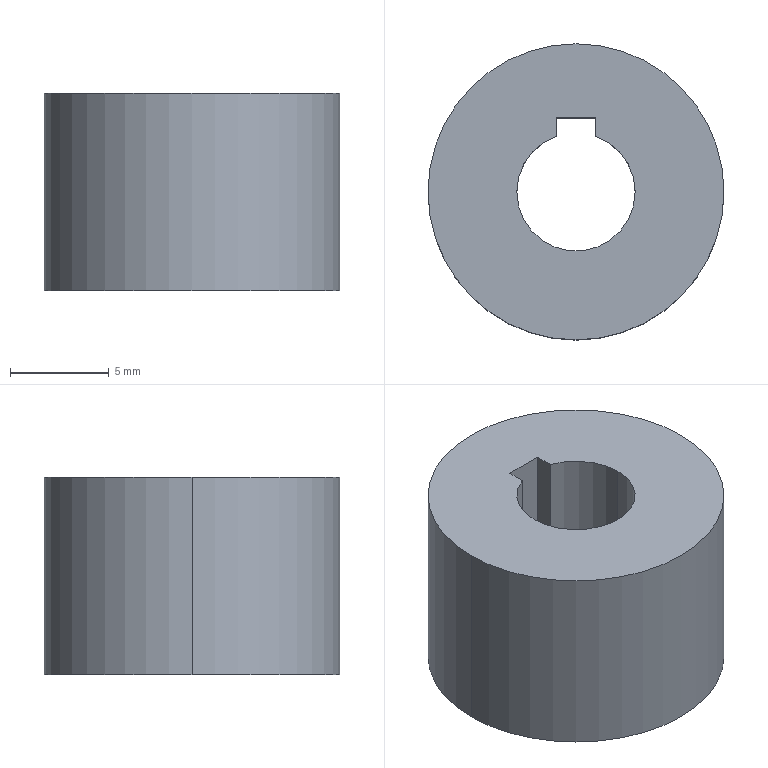Component | SolidWorks | SmallWheel-1 | 1 solid | 10 faces | box 15 x 15 x 10 mm | volume 1468 mm3 | cylinder 5 | plane 5 | commonest cylinder face diameters 6 x3 15 x2
build123d program:
from build123d import *

# Parameters (mm, degrees)
SKETCH1_R           = 7.5
SKETCH1_R_2         = 3
BOSS_EXTRUDE1_DEPTH = 10
SKETCH2_W           = 2
SKETCH2_H           = 1.5
CUT_EXTRUDE1_DEPTH  = 74.46


with BuildPart() as part:
    # Sketch1 → Boss-Extrude1 (new body)
    with BuildSketch(Plane.XY):
        with Locations((59.88, -20)):
            Circle(SKETCH1_R)
        with Locations((59.88, -20)):
            Circle(SKETCH1_R_2, mode=Mode.SUBTRACT)
    extrude(amount=-BOSS_EXTRUDE1_DEPTH)

    # Sketch2 → Cut-Extrude1 (cut, through all)
    with BuildSketch(Plane.XY):
        with Locations((59.88, -17)):
            Rectangle(SKETCH2_W, SKETCH2_H)
    extrude(amount=-CUT_EXTRUDE1_DEPTH, mode=Mode.SUBTRACT)


solid = part.part

# Placed as in the assembly
solid = solid.moved(Location((-11.374, -44.609, -195), (0, 0, 0)))
STEP:
#1=COLOUR_RGB('',0.7922,0.8196,0.9333);
#2=FILL_AREA_STYLE_COLOUR('',#1);
#3=FILL_AREA_STYLE('',(#2));
#4=SURFACE_STYLE_FILL_AREA(#3);
#5=SURFACE_SIDE_STYLE('',(#4));
#6=SURFACE_STYLE_USAGE(.BOTH.,#5);
#7=PRESENTATION_STYLE_ASSIGNMENT((#6));
#8=CARTESIAN_POINT('',(1.792,-2.544,-8.071));
#9=VERTEX_POINT('',#8);
#10=CARTESIAN_POINT('',(2.028,-2.544,-8.071));
#11=VERTEX_POINT('',#10);
#12=CARTESIAN_POINT('',(1.91,-2.544,-8.071));
#13=DIRECTION('',(0.,0.,1.));
#14=DIRECTION('',(1.,0.,0.));
#15=AXIS2_PLACEMENT_3D('',#12,#13,#14);
#16=CIRCLE('',#15,0.1181);
#17=EDGE_CURVE('',#9,#11,#16,.T.);
#18=ORIENTED_EDGE('',*,*,#17,.F.);
#19=CARTESIAN_POINT('',(1.792,-2.544,-7.677));
#20=VERTEX_POINT('',#19);
#21=CARTESIAN_POINT('',(1.792,-2.544,-8.071));
#22=DIRECTION('',(0.,0.,1.));
#23=VECTOR('',#22,39.37);
#24=LINE('',#21,#23);
#25=EDGE_CURVE('',#9,#20,#24,.T.);
#26=ORIENTED_EDGE('',*,*,#25,.T.);
#27=CARTESIAN_POINT('',(2.028,-2.544,-7.677));
#28=VERTEX_POINT('',#27);
#29=CARTESIAN_POINT('',(1.91,-2.544,-7.677));
#30=DIRECTION('',(0.,0.,1.));
#31=DIRECTION('',(1.,0.,0.));
#32=AXIS2_PLACEMENT_3D('',#29,#30,#31);
#33=CIRCLE('',#32,0.1181);
#34=EDGE_CURVE('',#20,#28,#33,.T.);
#35=ORIENTED_EDGE('',*,*,#34,.T.);
#36=CARTESIAN_POINT('',(2.028,-2.544,-8.071));
#37=DIRECTION('',(0.,0.,1.));
#38=VECTOR('',#37,39.37);
#39=LINE('',#36,#38);
#40=EDGE_CURVE('',#11,#28,#39,.T.);
#41=ORIENTED_EDGE('',*,*,#40,.F.);
#42=EDGE_LOOP('',(#18,#26,#35,#41));
#43=FACE_OUTER_BOUND('',#42,.T.);
#44=CARTESIAN_POINT('',(1.91,-2.544,-8.071));
#45=DIRECTION('',(0.,0.,1.));
#46=DIRECTION('',(1.,0.,0.));
#47=AXIS2_PLACEMENT_3D('',#44,#45,#46);
#48=CYLINDRICAL_SURFACE('',#47,0.1181);
#49=ADVANCED_FACE('',(#43),#48,.F.);
#50=CARTESIAN_POINT('',(1.949,-2.432,-8.071));
#51=VERTEX_POINT('',#50);
#52=CARTESIAN_POINT('',(1.91,-2.544,-8.071));
#53=DIRECTION('',(0.,0.,1.));
#54=DIRECTION('',(1.,0.,0.));
#55=AXIS2_PLACEMENT_3D('',#52,#53,#54);
#56=CIRCLE('',#55,0.1181);
#57=EDGE_CURVE('',#11,#51,#56,.T.);
#58=ORIENTED_EDGE('',*,*,#57,.F.);
#59=ORIENTED_EDGE('',*,*,#40,.T.);
#60=CARTESIAN_POINT('',(1.949,-2.432,-7.677));
#61=VERTEX_POINT('',#60);
#62=CARTESIAN_POINT('',(1.91,-2.544,-7.677));
#63=DIRECTION('',(0.,0.,1.));
#64=DIRECTION('',(1.,0.,0.));
#65=AXIS2_PLACEMENT_3D('',#62,#63,#64);
#66=CIRCLE('',#65,0.1181);
#67=EDGE_CURVE('',#28,#61,#66,.T.);
#68=ORIENTED_EDGE('',*,*,#67,.T.);
#69=CARTESIAN_POINT('',(1.949,-2.432,-8.071));
#70=DIRECTION('',(0.,0.,-1.));
#71=VECTOR('',#70,39.37);
#72=LINE('',#69,#71);
#73=EDGE_CURVE('',#61,#51,#72,.T.);
#74=ORIENTED_EDGE('',*,*,#73,.T.);
#75=EDGE_LOOP('',(#58,#59,#68,#74));
#76=FACE_OUTER_BOUND('',#75,.T.);
#77=CARTESIAN_POINT('',(1.91,-2.544,-8.071));
#78=DIRECTION('',(0.,0.,1.));
#79=DIRECTION('',(1.,0.,0.));
#80=AXIS2_PLACEMENT_3D('',#77,#78,#79);
#81=CYLINDRICAL_SURFACE('',#80,0.1181);
#82=ADVANCED_FACE('',(#76),#81,.F.);
#83=CARTESIAN_POINT('',(2.205,-2.544,-8.071));
#84=VERTEX_POINT('',#83);
#85=CARTESIAN_POINT('',(1.614,-2.544,-8.071));
#86=VERTEX_POINT('',#85);
#87=CARTESIAN_POINT('',(1.91,-2.544,-8.071));
#88=DIRECTION('',(0.,0.,1.));
#89=DIRECTION('',(1.,0.,0.));
#90=AXIS2_PLACEMENT_3D('',#87,#88,#89);
#91=CIRCLE('',#90,0.2953);
#92=EDGE_CURVE('',#84,#86,#91,.T.);
#93=ORIENTED_EDGE('',*,*,#92,.T.);
#94=CARTESIAN_POINT('',(1.614,-2.544,-7.677));
#95=VERTEX_POINT('',#94);
#96=CARTESIAN_POINT('',(1.614,-2.544,-8.071));
#97=DIRECTION('',(0.,0.,1.));
#98=VECTOR('',#97,39.37);
#99=LINE('',#96,#98);
#100=EDGE_CURVE('',#86,#95,#99,.T.);
#101=ORIENTED_EDGE('',*,*,#100,.T.);
#102=CARTESIAN_POINT('',(2.205,-2.544,-7.677));
#103=VERTEX_POINT('',#102);
#104=CARTESIAN_POINT('',(1.91,-2.544,-7.677));
#105=DIRECTION('',(0.,0.,1.));
#106=DIRECTION('',(1.,0.,0.));
#107=AXIS2_PLACEMENT_3D('',#104,#105,#106);
#108=CIRCLE('',#107,0.2953);
#109=EDGE_CURVE('',#103,#95,#108,.T.);
#110=ORIENTED_EDGE('',*,*,#109,.F.);
#111=CARTESIAN_POINT('',(2.205,-2.544,-8.071));
#112=DIRECTION('',(0.,0.,1.));
#113=VECTOR('',#112,39.37);
#114=LINE('',#111,#113);
#115=EDGE_CURVE('',#84,#103,#114,.T.);
#116=ORIENTED_EDGE('',*,*,#115,.F.);
#117=EDGE_LOOP('',(#93,#101,#110,#116));
#118=FACE_OUTER_BOUND('',#117,.T.);
#119=CARTESIAN_POINT('',(1.91,-2.544,-8.071));
#120=DIRECTION('',(0.,0.,1.));
#121=DIRECTION('',(1.,0.,0.));
#122=AXIS2_PLACEMENT_3D('',#119,#120,#121);
#123=CYLINDRICAL_SURFACE('',#122,0.2953);
#124=ADVANCED_FACE('',(#118),#123,.T.);
#125=ORIENTED_EDGE('',*,*,#100,.F.);
#126=CARTESIAN_POINT('',(1.91,-2.544,-8.071));
#127=DIRECTION('',(0.,0.,1.));
#128=DIRECTION('',(1.,0.,0.));
#129=AXIS2_PLACEMENT_3D('',#126,#127,#128);
#130=CIRCLE('',#129,0.2953);
#131=EDGE_CURVE('',#86,#84,#130,.T.);
#132=ORIENTED_EDGE('',*,*,#131,.T.);
#133=ORIENTED_EDGE('',*,*,#115,.T.);
#134=CARTESIAN_POINT('',(1.91,-2.544,-7.677));
#135=DIRECTION('',(0.,0.,1.));
#136=DIRECTION('',(1.,0.,0.));
#137=AXIS2_PLACEMENT_3D('',#134,#135,#136);
#138=CIRCLE('',#137,0.2953);
#139=EDGE_CURVE('',#95,#103,#138,.T.);
#140=ORIENTED_EDGE('',*,*,#139,.F.);
#141=EDGE_LOOP('',(#125,#132,#133,#140));
#142=FACE_OUTER_BOUND('',#141,.T.);
#143=CARTESIAN_POINT('',(1.91,-2.544,-8.071));
#144=DIRECTION('',(0.,0.,1.));
#145=DIRECTION('',(1.,0.,0.));
#146=AXIS2_PLACEMENT_3D('',#143,#144,#145);
#147=CYLINDRICAL_SURFACE('',#146,0.2953);
#148=ADVANCED_FACE('',(#142),#147,.T.);
#149=CARTESIAN_POINT('',(1.87,-2.432,-8.071));
#150=VERTEX_POINT('',#149);
#151=CARTESIAN_POINT('',(1.91,-2.544,-8.071));
#152=DIRECTION('',(0.,0.,1.));
#153=DIRECTION('',(1.,0.,0.));
#154=AXIS2_PLACEMENT_3D('',#151,#152,#153);
#155=CIRCLE('',#154,0.1181);
#156=EDGE_CURVE('',#150,#9,#155,.T.);
#157=ORIENTED_EDGE('',*,*,#156,.T.);
#158=ORIENTED_EDGE('',*,*,#17,.T.);
#159=ORIENTED_EDGE('',*,*,#57,.T.);
#160=CARTESIAN_POINT('',(1.949,-2.396,-8.071));
#161=VERTEX_POINT('',#160);
#162=CARTESIAN_POINT('',(1.949,-2.455,-8.071));
#163=DIRECTION('',(0.,1.,0.));
#164=VECTOR('',#163,39.37);
#165=LINE('',#162,#164);
#166=EDGE_CURVE('',#51,#161,#165,.T.);
#167=ORIENTED_EDGE('',*,*,#166,.T.);
#168=CARTESIAN_POINT('',(1.87,-2.396,-8.071));
#169=VERTEX_POINT('',#168);
#170=CARTESIAN_POINT('',(1.87,-2.396,-8.071));
#171=DIRECTION('',(-1.,0.,0.));
#172=VECTOR('',#171,39.37);
#173=LINE('',#170,#172);
#174=EDGE_CURVE('',#161,#169,#173,.T.);
#175=ORIENTED_EDGE('',*,*,#174,.T.);
#176=CARTESIAN_POINT('',(1.87,-2.455,-8.071));
#177=DIRECTION('',(0.,-1.,0.));
#178=VECTOR('',#177,39.37);
#179=LINE('',#176,#178);
#180=EDGE_CURVE('',#169,#150,#179,.T.);
#181=ORIENTED_EDGE('',*,*,#180,.T.);
#182=EDGE_LOOP('',(#157,#158,#159,#167,#175,#181));
#183=FACE_BOUND('',#182,.T.);
#184=ORIENTED_EDGE('',*,*,#92,.F.);
#185=ORIENTED_EDGE('',*,*,#131,.F.);
#186=EDGE_LOOP('',(#184,#185));
#187=FACE_OUTER_BOUND('',#186,.T.);
#188=CARTESIAN_POINT('',(1.91,-2.544,-8.071));
#189=DIRECTION('',(0.,0.,1.));
#190=DIRECTION('',(1.,0.,0.));
#191=AXIS2_PLACEMENT_3D('',#188,#189,#190);
#192=PLANE('',#191);
#193=ADVANCED_FACE('',(#183,#187),#192,.F.);
#194=CARTESIAN_POINT('',(1.949,-2.396,-7.677));
#195=VERTEX_POINT('',#194);
#196=CARTESIAN_POINT('',(1.949,-2.455,-7.677));
#197=DIRECTION('',(0.,1.,0.));
#198=VECTOR('',#197,39.37);
#199=LINE('',#196,#198);
#200=EDGE_CURVE('',#61,#195,#199,.T.);
#201=ORIENTED_EDGE('',*,*,#200,.F.);
#202=ORIENTED_EDGE('',*,*,#67,.F.);
#203=ORIENTED_EDGE('',*,*,#34,.F.);
#204=CARTESIAN_POINT('',(1.87,-2.432,-7.677));
#205=VERTEX_POINT('',#204);
#206=CARTESIAN_POINT('',(1.91,-2.544,-7.677));
#207=DIRECTION('',(0.,0.,1.));
#208=DIRECTION('',(1.,0.,0.));
#209=AXIS2_PLACEMENT_3D('',#206,#207,#208);
#210=CIRCLE('',#209,0.1181);
#211=EDGE_CURVE('',#205,#20,#210,.T.);
#212=ORIENTED_EDGE('',*,*,#211,.F.);
#213=CARTESIAN_POINT('',(1.87,-2.396,-7.677));
#214=VERTEX_POINT('',#213);
#215=CARTESIAN_POINT('',(1.87,-2.455,-7.677));
#216=DIRECTION('',(0.,-1.,0.));
#217=VECTOR('',#216,39.37);
#218=LINE('',#215,#217);
#219=EDGE_CURVE('',#214,#205,#218,.T.);
#220=ORIENTED_EDGE('',*,*,#219,.F.);
#221=CARTESIAN_POINT('',(1.87,-2.396,-7.677));
#222=DIRECTION('',(-1.,0.,0.));
#223=VECTOR('',#222,39.37);
#224=LINE('',#221,#223);
#225=EDGE_CURVE('',#195,#214,#224,.T.);
#226=ORIENTED_EDGE('',*,*,#225,.F.);
#227=EDGE_LOOP('',(#201,#202,#203,#212,#220,#226));
#228=FACE_BOUND('',#227,.T.);
#229=ORIENTED_EDGE('',*,*,#109,.T.);
#230=ORIENTED_EDGE('',*,*,#139,.T.);
#231=EDGE_LOOP('',(#229,#230));
#232=FACE_OUTER_BOUND('',#231,.T.);
#233=CARTESIAN_POINT('',(1.91,-2.544,-7.677));
#234=DIRECTION('',(0.,0.,1.));
#235=DIRECTION('',(1.,0.,0.));
#236=AXIS2_PLACEMENT_3D('',#233,#234,#235);
#237=PLANE('',#236);
#238=ADVANCED_FACE('',(#228,#232),#237,.T.);
#239=ORIENTED_EDGE('',*,*,#25,.F.);
#240=ORIENTED_EDGE('',*,*,#156,.F.);
#241=CARTESIAN_POINT('',(1.87,-2.432,-8.071));
#242=DIRECTION('',(0.,0.,1.));
#243=VECTOR('',#242,39.37);
#244=LINE('',#241,#243);
#245=EDGE_CURVE('',#150,#205,#244,.T.);
#246=ORIENTED_EDGE('',*,*,#245,.T.);
#247=ORIENTED_EDGE('',*,*,#211,.T.);
#248=EDGE_LOOP('',(#239,#240,#246,#247));
#249=FACE_OUTER_BOUND('',#248,.T.);
#250=CARTESIAN_POINT('',(1.91,-2.544,-8.071));
#251=DIRECTION('',(0.,0.,1.));
#252=DIRECTION('',(1.,0.,0.));
#253=AXIS2_PLACEMENT_3D('',#250,#251,#252);
#254=CYLINDRICAL_SURFACE('',#253,0.1181);
#255=ADVANCED_FACE('',(#249),#254,.F.);
#256=ORIENTED_EDGE('',*,*,#200,.T.);
#257=CARTESIAN_POINT('',(1.949,-2.396,-8.071));
#258=DIRECTION('',(0.,0.,1.));
#259=VECTOR('',#258,39.37);
#260=LINE('',#257,#259);
#261=EDGE_CURVE('',#161,#195,#260,.T.);
#262=ORIENTED_EDGE('',*,*,#261,.F.);
#263=ORIENTED_EDGE('',*,*,#166,.F.);
#264=ORIENTED_EDGE('',*,*,#73,.F.);
#265=EDGE_LOOP('',(#256,#262,#263,#264));
#266=FACE_OUTER_BOUND('',#265,.T.);
#267=CARTESIAN_POINT('',(1.949,-2.455,-8.071));
#268=DIRECTION('',(1.,0.,0.));
#269=DIRECTION('',(0.,0.,-1.));
#270=AXIS2_PLACEMENT_3D('',#267,#268,#269);
#271=PLANE('',#270);
#272=ADVANCED_FACE('',(#266),#271,.F.);
#273=ORIENTED_EDGE('',*,*,#180,.F.);
#274=CARTESIAN_POINT('',(1.87,-2.396,-8.071));
#275=DIRECTION('',(0.,0.,1.));
#276=VECTOR('',#275,39.37);
#277=LINE('',#274,#276);
#278=EDGE_CURVE('',#169,#214,#277,.T.);
#279=ORIENTED_EDGE('',*,*,#278,.T.);
#280=ORIENTED_EDGE('',*,*,#219,.T.);
#281=ORIENTED_EDGE('',*,*,#245,.F.);
#282=EDGE_LOOP('',(#273,#279,#280,#281));
#283=FACE_OUTER_BOUND('',#282,.T.);
#284=CARTESIAN_POINT('',(1.87,-2.455,-8.071));
#285=DIRECTION('',(-1.,0.,0.));
#286=DIRECTION('',(0.,0.,1.));
#287=AXIS2_PLACEMENT_3D('',#284,#285,#286);
#288=PLANE('',#287);
#289=ADVANCED_FACE('',(#283),#288,.F.);
#290=ORIENTED_EDGE('',*,*,#225,.T.);
#291=ORIENTED_EDGE('',*,*,#278,.F.);
#292=ORIENTED_EDGE('',*,*,#174,.F.);
#293=ORIENTED_EDGE('',*,*,#261,.T.);
#294=EDGE_LOOP('',(#290,#291,#292,#293));
#295=FACE_OUTER_BOUND('',#294,.T.);
#296=CARTESIAN_POINT('',(1.87,-2.396,-8.071));
#297=DIRECTION('',(0.,1.,0.));
#298=DIRECTION('',(0.,0.,1.));
#299=AXIS2_PLACEMENT_3D('',#296,#297,#298);
#300=PLANE('',#299);
#301=ADVANCED_FACE('',(#295),#300,.F.);
#302=CLOSED_SHELL('',(#49,#82,#124,#148,#193,#238,#255,#272,#289,#301));
#303=MANIFOLD_SOLID_BREP('',#302);
#304=STYLED_ITEM('',(#7),#303);
#305=PRESENTATION_LAYER_ASSIGNMENT('','',(#304));
#306=CARTESIAN_POINT('',(0.,0.,0.));
#307=DIRECTION('',(0.,0.,1.));
#308=DIRECTION('',(1.,0.,0.));
#309=AXIS2_PLACEMENT_3D('',#306,#307,#308);
#310=(LENGTH_UNIT()NAMED_UNIT(*)SI_UNIT($,.METRE.));
#311=LENGTH_MEASURE_WITH_UNIT(LENGTH_MEASURE(0.0254),#310);
#312=DIMENSIONAL_EXPONENTS(1.,0.,0.,0.,0.,0.,0.);
#313=(CONVERSION_BASED_UNIT('',#311)LENGTH_UNIT()NAMED_UNIT(#312));
#314=UNCERTAINTY_MEASURE_WITH_UNIT(LENGTH_MEASURE(0.00001),#313,'','');
#315=(NAMED_UNIT(*)PLANE_ANGLE_UNIT()SI_UNIT($,.RADIAN.));
#316=(NAMED_UNIT(*)SI_UNIT($,.STERADIAN.)SOLID_ANGLE_UNIT());
#317=(GEOMETRIC_REPRESENTATION_CONTEXT(3)GLOBAL_UNCERTAINTY_ASSIGNED_CONTEXT((#314))GLOBAL_UNIT_ASSIGNED_CONTEXT((#313,#315,#316))REPRESENTATION_CONTEXT('',''));
#318=ADVANCED_BREP_SHAPE_REPRESENTATION('',(#303,#309),#317);
#319=(LENGTH_UNIT()NAMED_UNIT(*)SI_UNIT($,.METRE.));
#320=LENGTH_MEASURE_WITH_UNIT(LENGTH_MEASURE(0.0254),#319);
#321=DIMENSIONAL_EXPONENTS(1.,0.,0.,0.,0.,0.,0.);
#322=(CONVERSION_BASED_UNIT('',#320)LENGTH_UNIT()NAMED_UNIT(#321));
#323=UNCERTAINTY_MEASURE_WITH_UNIT(LENGTH_MEASURE(0.00001),#322,'','');
#324=(NAMED_UNIT(*)PLANE_ANGLE_UNIT()SI_UNIT($,.RADIAN.));
#325=(NAMED_UNIT(*)SI_UNIT($,.STERADIAN.)SOLID_ANGLE_UNIT());
#326=(GEOMETRIC_REPRESENTATION_CONTEXT(3)GLOBAL_UNCERTAINTY_ASSIGNED_CONTEXT((#323))GLOBAL_UNIT_ASSIGNED_CONTEXT((#322,#324,#325))REPRESENTATION_CONTEXT('',''));
#327=MECHANICAL_DESIGN_GEOMETRIC_PRESENTATION_REPRESENTATION('',(#304),#326);